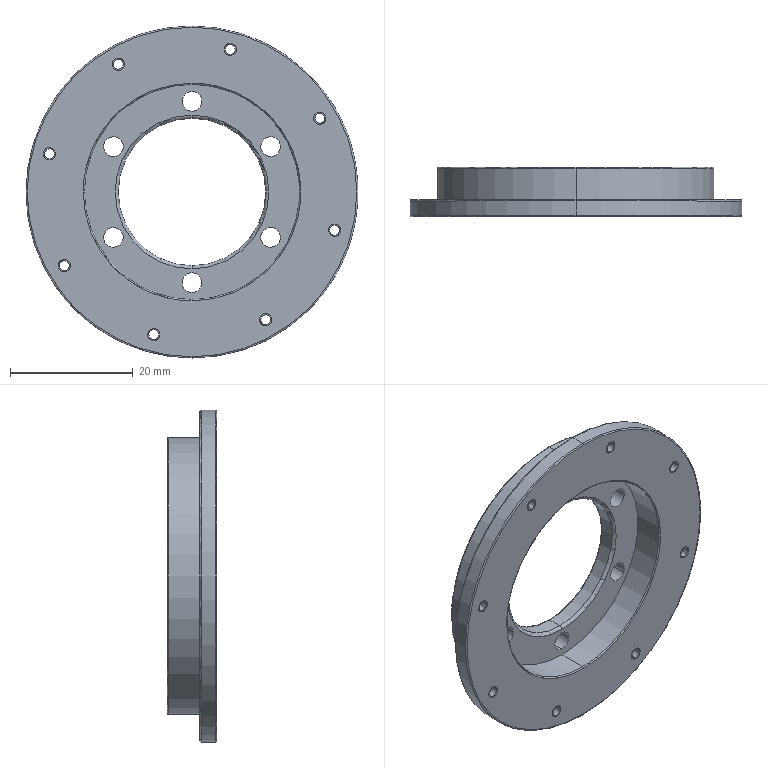CAM job | Mastercam | mm | 4 operations | part box 54 x 8 x 54
1. Drill/Counterbore | 7 - 4 倒角刀
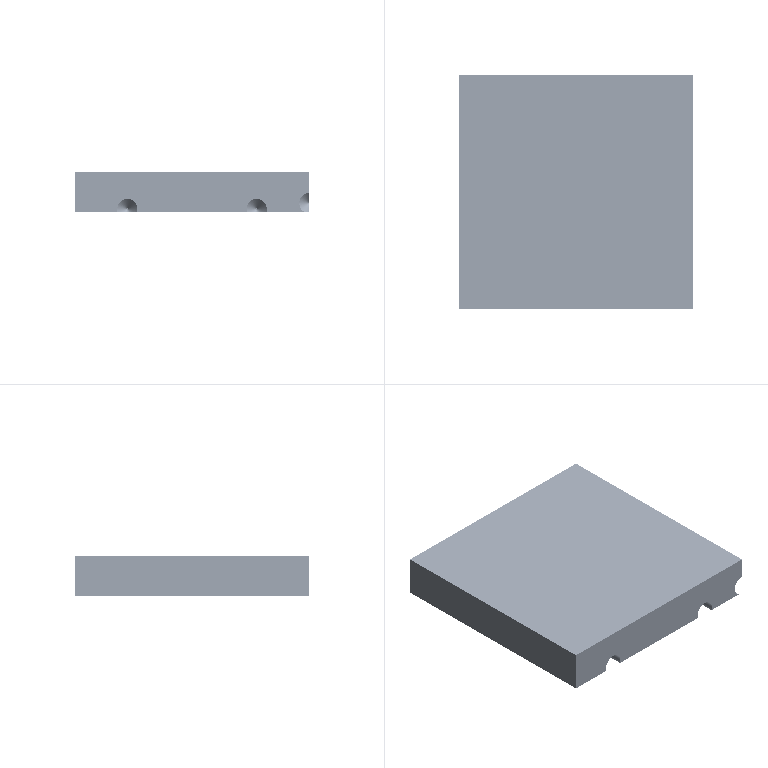2. 2D High Speed (2D Area Mill) | 8 - 8 平铣刀
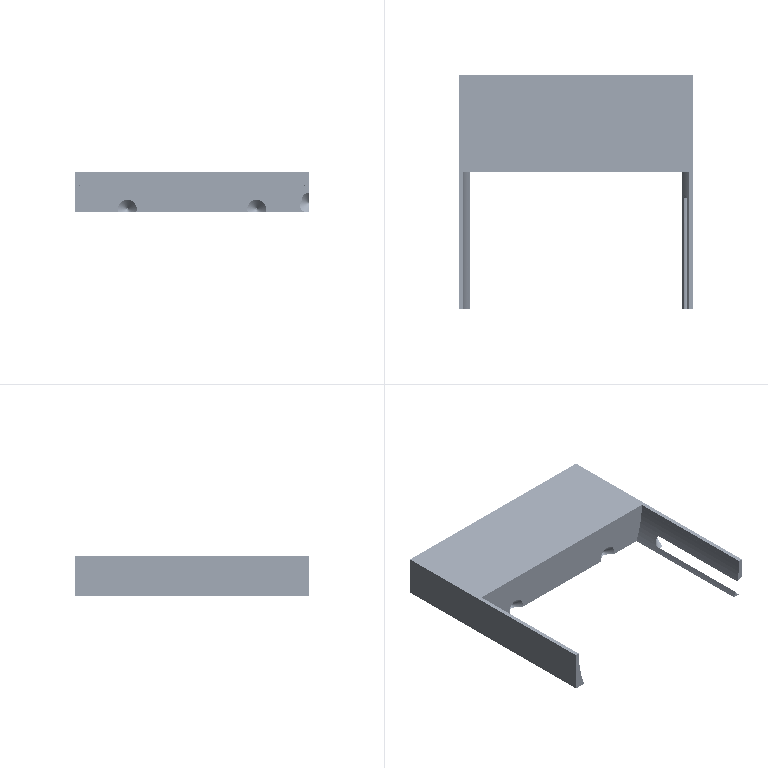3. Contour (2D) | 8 - 8 平铣刀
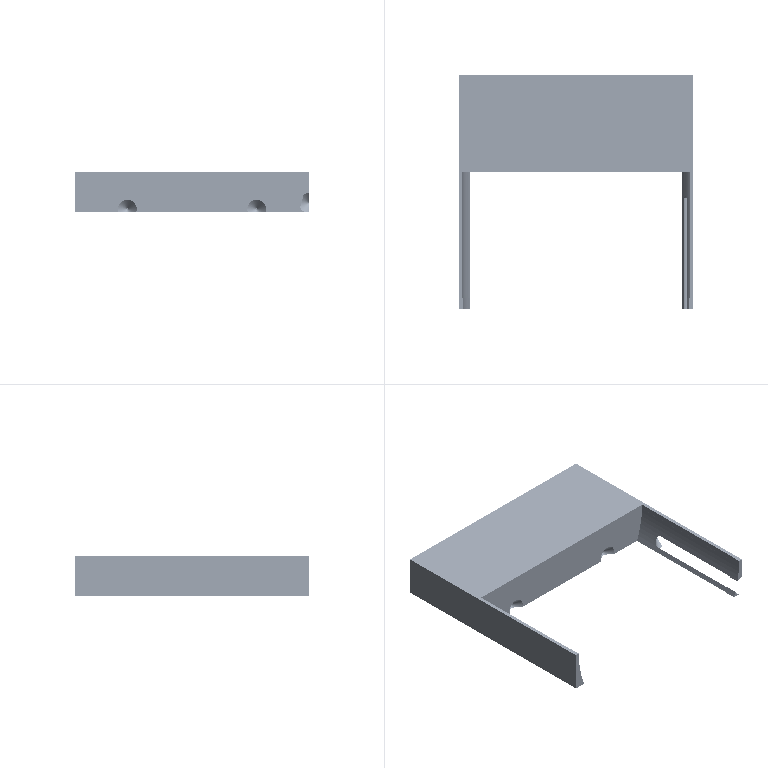4. Contour (2D chamfer) | 7 - 4 倒角刀